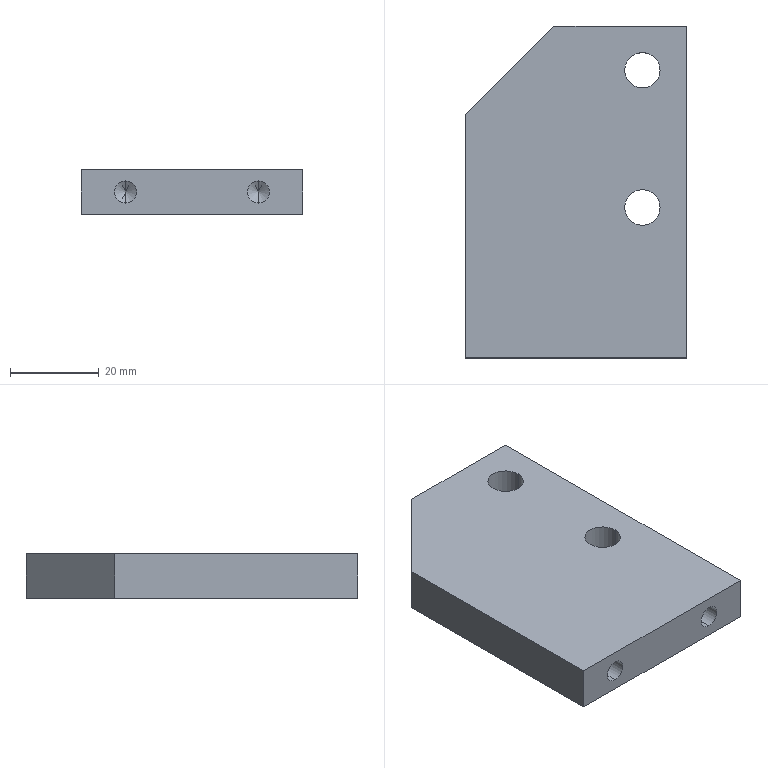Component | SolidWorks | JL001-05-05-002-1 | 1 solid | 19 faces | box 50 x 75 x 10 mm | volume 33886 mm3 | cylinder 8 | plane 7 | cone 4 | commonest cylinder face diameters 5 x4 8 x4
build123d program:
from build123d import *

# Parameters (mm, degrees)
SKETCH1_W             = 50
SKETCH1_H             = 75
BOSS_EXTRUDE1_DEPTH   = 5
M8X1_0_TAPPED_HOLE1_D = 8
M6_TAPPED_HOLE1_D     = 5
M6_TAPPED_HOLE1_DEPTH = 15
M6_TAPPED_HOLE1_TIP   = 1.502
CHAMFER1_SIZE         = 20


with BuildPart() as part:
    # Sketch1 → Boss-Extrude1 (new, symmetric)
    with BuildSketch(Plane.XY):
        Rectangle(SKETCH1_W, SKETCH1_H)
    extrude(amount=BOSS_EXTRUDE1_DEPTH, both=True)

    # M8x1.0 Tapped Hole1 (through all)
    with Locations(Plane.XY.offset(5)):
        with Locations((15, 27.5), (15, -3.5)):
            Hole(M8X1_0_TAPPED_HOLE1_D / 2)

    # M6 Tapped Hole1
    with Locations(Plane(origin=(0, -37.5, 0), x_dir=(-1, 0, 0), z_dir=(0, -1, 0))):
        with Locations((15, 0), (-15, 0)):
            Hole(M6_TAPPED_HOLE1_D / 2, depth=M6_TAPPED_HOLE1_DEPTH)
            with Locations((0, 0, -(M6_TAPPED_HOLE1_DEPTH + M6_TAPPED_HOLE1_TIP / 2))):  # 118° drill point
                Cone(0, M6_TAPPED_HOLE1_D / 2, M6_TAPPED_HOLE1_TIP, mode=Mode.SUBTRACT)

    # Chamfer1
    chamfer1_edges = [part.edges().sort_by_distance(p)[0] for p in [
        (-25, 37.5, 0),
    ]]
    chamfer(chamfer1_edges, length=CHAMFER1_SIZE)


solid = part.part

# Placed as in the assembly
solid = solid.moved(Location((0, 0, 137.5), (0, 0, 0)))
STEP:
#1=CARTESIAN_POINT('',(-0.5906,-0.8858,5.512));
#2=VERTEX_POINT('',#1);
#3=CARTESIAN_POINT('',(-0.5906,-0.8858,5.315));
#4=VERTEX_POINT('',#3);
#5=CARTESIAN_POINT('',(-0.5906,-0.8858,5.413));
#6=DIRECTION('',(0.,-1.,0.));
#7=DIRECTION('',(0.,0.,-1.));
#8=AXIS2_PLACEMENT_3D('',#5,#6,#7);
#9=CIRCLE('',#8,0.09843);
#10=EDGE_CURVE('',#2,#4,#9,.T.);
#11=ORIENTED_EDGE('',*,*,#10,.F.);
#12=CARTESIAN_POINT('',(-0.5906,-1.476,5.512));
#13=VERTEX_POINT('',#12);
#14=CARTESIAN_POINT('',(-0.5906,-1.476,5.512));
#15=DIRECTION('',(0.,-1.,0.));
#16=VECTOR('',#15,39.37);
#17=LINE('',#14,#16);
#18=EDGE_CURVE('',#2,#13,#17,.T.);
#19=ORIENTED_EDGE('',*,*,#18,.T.);
#20=CARTESIAN_POINT('',(-0.5906,-1.476,5.315));
#21=VERTEX_POINT('',#20);
#22=CARTESIAN_POINT('',(-0.5906,-1.476,5.413));
#23=DIRECTION('',(0.,-1.,0.));
#24=DIRECTION('',(0.,0.,-1.));
#25=AXIS2_PLACEMENT_3D('',#22,#23,#24);
#26=CIRCLE('',#25,0.09843);
#27=EDGE_CURVE('',#13,#21,#26,.T.);
#28=ORIENTED_EDGE('',*,*,#27,.T.);
#29=CARTESIAN_POINT('',(-0.5906,-1.476,5.315));
#30=DIRECTION('',(0.,-1.,0.));
#31=VECTOR('',#30,39.37);
#32=LINE('',#29,#31);
#33=EDGE_CURVE('',#4,#21,#32,.T.);
#34=ORIENTED_EDGE('',*,*,#33,.F.);
#35=EDGE_LOOP('',(#11,#19,#28,#34));
#36=FACE_OUTER_BOUND('',#35,.T.);
#37=CARTESIAN_POINT('',(-0.5906,-1.476,5.413));
#38=DIRECTION('',(0.,-1.,0.));
#39=DIRECTION('',(0.,0.,-1.));
#40=AXIS2_PLACEMENT_3D('',#37,#38,#39);
#41=CYLINDRICAL_SURFACE('',#40,0.09843);
#42=ADVANCED_FACE('',(#36),#41,.F.);
#43=CARTESIAN_POINT('',(-0.5906,-0.8267,5.413));
#44=VERTEX_POINT('',#43);
#45=CARTESIAN_POINT('',(-0.5906,-0.8858,5.315));
#46=DIRECTION('',(0.,-0.515,-0.8572));
#47=VECTOR('',#46,39.37);
#48=LINE('',#45,#47);
#49=EDGE_CURVE('',#44,#4,#48,.T.);
#50=ORIENTED_EDGE('',*,*,#49,.F.);
#51=CARTESIAN_POINT('',(-0.5906,-0.8858,5.512));
#52=DIRECTION('',(0.,-0.515,0.8572));
#53=VECTOR('',#52,39.37);
#54=LINE('',#51,#53);
#55=EDGE_CURVE('',#44,#2,#54,.T.);
#56=ORIENTED_EDGE('',*,*,#55,.T.);
#57=ORIENTED_EDGE('',*,*,#10,.T.);
#58=EDGE_LOOP('',(#50,#56,#57));
#59=FACE_OUTER_BOUND('',#58,.T.);
#60=CARTESIAN_POINT('',(-0.5906,-0.8858,5.413));
#61=DIRECTION('',(0.,-1.,0.));
#62=DIRECTION('',(0.,0.,-1.));
#63=AXIS2_PLACEMENT_3D('',#60,#61,#62);
#64=CONICAL_SURFACE('',#63,0.09843,1.03);
#65=ADVANCED_FACE('',(#59),#64,.F.);
#66=CARTESIAN_POINT('',(0.5906,-0.8858,5.512));
#67=VERTEX_POINT('',#66);
#68=CARTESIAN_POINT('',(0.5906,-0.8858,5.315));
#69=VERTEX_POINT('',#68);
#70=CARTESIAN_POINT('',(0.5906,-0.8858,5.413));
#71=DIRECTION('',(0.,-1.,0.));
#72=DIRECTION('',(0.,0.,-1.));
#73=AXIS2_PLACEMENT_3D('',#70,#71,#72);
#74=CIRCLE('',#73,0.09843);
#75=EDGE_CURVE('',#67,#69,#74,.T.);
#76=ORIENTED_EDGE('',*,*,#75,.F.);
#77=CARTESIAN_POINT('',(0.5906,-1.476,5.512));
#78=VERTEX_POINT('',#77);
#79=CARTESIAN_POINT('',(0.5906,-1.476,5.512));
#80=DIRECTION('',(0.,-1.,0.));
#81=VECTOR('',#80,39.37);
#82=LINE('',#79,#81);
#83=EDGE_CURVE('',#67,#78,#82,.T.);
#84=ORIENTED_EDGE('',*,*,#83,.T.);
#85=CARTESIAN_POINT('',(0.5906,-1.476,5.315));
#86=VERTEX_POINT('',#85);
#87=CARTESIAN_POINT('',(0.5906,-1.476,5.413));
#88=DIRECTION('',(0.,-1.,0.));
#89=DIRECTION('',(0.,0.,-1.));
#90=AXIS2_PLACEMENT_3D('',#87,#88,#89);
#91=CIRCLE('',#90,0.09843);
#92=EDGE_CURVE('',#78,#86,#91,.T.);
#93=ORIENTED_EDGE('',*,*,#92,.T.);
#94=CARTESIAN_POINT('',(0.5906,-1.476,5.315));
#95=DIRECTION('',(0.,-1.,0.));
#96=VECTOR('',#95,39.37);
#97=LINE('',#94,#96);
#98=EDGE_CURVE('',#69,#86,#97,.T.);
#99=ORIENTED_EDGE('',*,*,#98,.F.);
#100=EDGE_LOOP('',(#76,#84,#93,#99));
#101=FACE_OUTER_BOUND('',#100,.T.);
#102=CARTESIAN_POINT('',(0.5906,-1.476,5.413));
#103=DIRECTION('',(0.,-1.,0.));
#104=DIRECTION('',(0.,0.,-1.));
#105=AXIS2_PLACEMENT_3D('',#102,#103,#104);
#106=CYLINDRICAL_SURFACE('',#105,0.09843);
#107=ADVANCED_FACE('',(#101),#106,.F.);
#108=CARTESIAN_POINT('',(0.5906,-0.8267,5.413));
#109=VERTEX_POINT('',#108);
#110=CARTESIAN_POINT('',(0.5906,-0.8858,5.315));
#111=DIRECTION('',(0.,-0.515,-0.8572));
#112=VECTOR('',#111,39.37);
#113=LINE('',#110,#112);
#114=EDGE_CURVE('',#109,#69,#113,.T.);
#115=ORIENTED_EDGE('',*,*,#114,.F.);
#116=CARTESIAN_POINT('',(0.5906,-0.8858,5.512));
#117=DIRECTION('',(0.,-0.515,0.8572));
#118=VECTOR('',#117,39.37);
#119=LINE('',#116,#118);
#120=EDGE_CURVE('',#109,#67,#119,.T.);
#121=ORIENTED_EDGE('',*,*,#120,.T.);
#122=ORIENTED_EDGE('',*,*,#75,.T.);
#123=EDGE_LOOP('',(#115,#121,#122));
#124=FACE_OUTER_BOUND('',#123,.T.);
#125=CARTESIAN_POINT('',(0.5906,-0.8858,5.413));
#126=DIRECTION('',(0.,-1.,0.));
#127=DIRECTION('',(0.,0.,-1.));
#128=AXIS2_PLACEMENT_3D('',#125,#126,#127);
#129=CONICAL_SURFACE('',#128,0.09843,1.03);
#130=ADVANCED_FACE('',(#124),#129,.F.);
#131=CARTESIAN_POINT('',(0.4331,1.083,5.217));
#132=VERTEX_POINT('',#131);
#133=CARTESIAN_POINT('',(0.748,1.083,5.217));
#134=VERTEX_POINT('',#133);
#135=CARTESIAN_POINT('',(0.5906,1.083,5.217));
#136=DIRECTION('',(0.,0.,1.));
#137=DIRECTION('',(1.,0.,0.));
#138=AXIS2_PLACEMENT_3D('',#135,#136,#137);
#139=CIRCLE('',#138,0.1575);
#140=EDGE_CURVE('',#132,#134,#139,.T.);
#141=ORIENTED_EDGE('',*,*,#140,.F.);
#142=CARTESIAN_POINT('',(0.4331,1.083,5.61));
#143=VERTEX_POINT('',#142);
#144=CARTESIAN_POINT('',(0.4331,1.083,5.61));
#145=DIRECTION('',(0.,0.,1.));
#146=VECTOR('',#145,39.37);
#147=LINE('',#144,#146);
#148=EDGE_CURVE('',#132,#143,#147,.T.);
#149=ORIENTED_EDGE('',*,*,#148,.T.);
#150=CARTESIAN_POINT('',(0.748,1.083,5.61));
#151=VERTEX_POINT('',#150);
#152=CARTESIAN_POINT('',(0.5906,1.083,5.61));
#153=DIRECTION('',(0.,0.,1.));
#154=DIRECTION('',(1.,0.,0.));
#155=AXIS2_PLACEMENT_3D('',#152,#153,#154);
#156=CIRCLE('',#155,0.1575);
#157=EDGE_CURVE('',#143,#151,#156,.T.);
#158=ORIENTED_EDGE('',*,*,#157,.T.);
#159=CARTESIAN_POINT('',(0.748,1.083,5.61));
#160=DIRECTION('',(0.,0.,1.));
#161=VECTOR('',#160,39.37);
#162=LINE('',#159,#161);
#163=EDGE_CURVE('',#134,#151,#162,.T.);
#164=ORIENTED_EDGE('',*,*,#163,.F.);
#165=EDGE_LOOP('',(#141,#149,#158,#164));
#166=FACE_OUTER_BOUND('',#165,.T.);
#167=CARTESIAN_POINT('',(0.5906,1.083,5.61));
#168=DIRECTION('',(0.,0.,1.));
#169=DIRECTION('',(1.,0.,0.));
#170=AXIS2_PLACEMENT_3D('',#167,#168,#169);
#171=CYLINDRICAL_SURFACE('',#170,0.1575);
#172=ADVANCED_FACE('',(#166),#171,.F.);
#173=CARTESIAN_POINT('',(0.4331,-0.1378,5.217));
#174=VERTEX_POINT('',#173);
#175=CARTESIAN_POINT('',(0.748,-0.1378,5.217));
#176=VERTEX_POINT('',#175);
#177=CARTESIAN_POINT('',(0.5906,-0.1378,5.217));
#178=DIRECTION('',(0.,0.,1.));
#179=DIRECTION('',(1.,0.,0.));
#180=AXIS2_PLACEMENT_3D('',#177,#178,#179);
#181=CIRCLE('',#180,0.1575);
#182=EDGE_CURVE('',#174,#176,#181,.T.);
#183=ORIENTED_EDGE('',*,*,#182,.F.);
#184=CARTESIAN_POINT('',(0.4331,-0.1378,5.61));
#185=VERTEX_POINT('',#184);
#186=CARTESIAN_POINT('',(0.4331,-0.1378,5.61));
#187=DIRECTION('',(0.,0.,1.));
#188=VECTOR('',#187,39.37);
#189=LINE('',#186,#188);
#190=EDGE_CURVE('',#174,#185,#189,.T.);
#191=ORIENTED_EDGE('',*,*,#190,.T.);
#192=CARTESIAN_POINT('',(0.748,-0.1378,5.61));
#193=VERTEX_POINT('',#192);
#194=CARTESIAN_POINT('',(0.5906,-0.1378,5.61));
#195=DIRECTION('',(0.,0.,1.));
#196=DIRECTION('',(1.,0.,0.));
#197=AXIS2_PLACEMENT_3D('',#194,#195,#196);
#198=CIRCLE('',#197,0.1575);
#199=EDGE_CURVE('',#185,#193,#198,.T.);
#200=ORIENTED_EDGE('',*,*,#199,.T.);
#201=CARTESIAN_POINT('',(0.748,-0.1378,5.61));
#202=DIRECTION('',(0.,0.,1.));
#203=VECTOR('',#202,39.37);
#204=LINE('',#201,#203);
#205=EDGE_CURVE('',#176,#193,#204,.T.);
#206=ORIENTED_EDGE('',*,*,#205,.F.);
#207=EDGE_LOOP('',(#183,#191,#200,#206));
#208=FACE_OUTER_BOUND('',#207,.T.);
#209=CARTESIAN_POINT('',(0.5906,-0.1378,5.61));
#210=DIRECTION('',(0.,0.,1.));
#211=DIRECTION('',(1.,0.,0.));
#212=AXIS2_PLACEMENT_3D('',#209,#210,#211);
#213=CYLINDRICAL_SURFACE('',#212,0.1575);
#214=ADVANCED_FACE('',(#208),#213,.F.);
#215=CARTESIAN_POINT('',(0.9843,-1.476,5.217));
#216=VERTEX_POINT('',#215);
#217=CARTESIAN_POINT('',(0.9843,1.476,5.217));
#218=VERTEX_POINT('',#217);
#219=CARTESIAN_POINT('',(0.9843,1.476,5.217));
#220=DIRECTION('',(-0.,1.,0.));
#221=VECTOR('',#220,39.37);
#222=LINE('',#219,#221);
#223=EDGE_CURVE('',#216,#218,#222,.T.);
#224=ORIENTED_EDGE('',*,*,#223,.T.);
#225=CARTESIAN_POINT('',(0.9843,1.476,5.61));
#226=VERTEX_POINT('',#225);
#227=CARTESIAN_POINT('',(0.9843,1.476,5.61));
#228=DIRECTION('',(0.,0.,-1.));
#229=VECTOR('',#228,39.37);
#230=LINE('',#227,#229);
#231=EDGE_CURVE('',#226,#218,#230,.T.);
#232=ORIENTED_EDGE('',*,*,#231,.F.);
#233=CARTESIAN_POINT('',(0.9843,-1.476,5.61));
#234=VERTEX_POINT('',#233);
#235=CARTESIAN_POINT('',(0.9843,1.476,5.61));
#236=DIRECTION('',(-0.,1.,0.));
#237=VECTOR('',#236,39.37);
#238=LINE('',#235,#237);
#239=EDGE_CURVE('',#234,#226,#238,.T.);
#240=ORIENTED_EDGE('',*,*,#239,.F.);
#241=CARTESIAN_POINT('',(0.9843,-1.476,5.61));
#242=DIRECTION('',(0.,0.,-1.));
#243=VECTOR('',#242,39.37);
#244=LINE('',#241,#243);
#245=EDGE_CURVE('',#234,#216,#244,.T.);
#246=ORIENTED_EDGE('',*,*,#245,.T.);
#247=EDGE_LOOP('',(#224,#232,#240,#246));
#248=FACE_OUTER_BOUND('',#247,.T.);
#249=CARTESIAN_POINT('',(0.9843,1.476,5.61));
#250=DIRECTION('',(-1.,-0.,0.));
#251=DIRECTION('',(0.,-1.,0.));
#252=AXIS2_PLACEMENT_3D('',#249,#250,#251);
#253=PLANE('',#252);
#254=ADVANCED_FACE('',(#248),#253,.F.);
#255=CARTESIAN_POINT('',(-0.1969,1.476,5.217));
#256=VERTEX_POINT('',#255);
#257=CARTESIAN_POINT('',(-0.9843,1.476,5.217));
#258=DIRECTION('',(-1.,0.,0.));
#259=VECTOR('',#258,39.37);
#260=LINE('',#257,#259);
#261=EDGE_CURVE('',#218,#256,#260,.T.);
#262=ORIENTED_EDGE('',*,*,#261,.T.);
#263=CARTESIAN_POINT('',(-0.1969,1.476,5.61));
#264=VERTEX_POINT('',#263);
#265=CARTESIAN_POINT('',(-0.1969,1.476,5.61));
#266=DIRECTION('',(0.,0.,1.));
#267=VECTOR('',#266,39.37);
#268=LINE('',#265,#267);
#269=EDGE_CURVE('',#256,#264,#268,.T.);
#270=ORIENTED_EDGE('',*,*,#269,.T.);
#271=CARTESIAN_POINT('',(-0.9843,1.476,5.61));
#272=DIRECTION('',(-1.,0.,0.));
#273=VECTOR('',#272,39.37);
#274=LINE('',#271,#273);
#275=EDGE_CURVE('',#226,#264,#274,.T.);
#276=ORIENTED_EDGE('',*,*,#275,.F.);
#277=ORIENTED_EDGE('',*,*,#231,.T.);
#278=EDGE_LOOP('',(#262,#270,#276,#277));
#279=FACE_OUTER_BOUND('',#278,.T.);
#280=CARTESIAN_POINT('',(-0.9843,1.476,5.61));
#281=DIRECTION('',(0.,-1.,0.));
#282=DIRECTION('',(0.,0.,-1.));
#283=AXIS2_PLACEMENT_3D('',#280,#281,#282);
#284=PLANE('',#283);
#285=ADVANCED_FACE('',(#279),#284,.F.);
#286=CARTESIAN_POINT('',(-0.9843,0.689,5.61));
#287=VERTEX_POINT('',#286);
#288=CARTESIAN_POINT('',(-0.9843,-1.476,5.61));
#289=VERTEX_POINT('',#288);
#290=CARTESIAN_POINT('',(-0.9843,1.476,5.61));
#291=DIRECTION('',(0.,-1.,0.));
#292=VECTOR('',#291,39.37);
#293=LINE('',#290,#292);
#294=EDGE_CURVE('',#287,#289,#293,.T.);
#295=ORIENTED_EDGE('',*,*,#294,.F.);
#296=CARTESIAN_POINT('',(-0.9843,0.689,5.217));
#297=VERTEX_POINT('',#296);
#298=CARTESIAN_POINT('',(-0.9843,0.689,5.61));
#299=DIRECTION('',(0.,0.,-1.));
#300=VECTOR('',#299,39.37);
#301=LINE('',#298,#300);
#302=EDGE_CURVE('',#287,#297,#301,.T.);
#303=ORIENTED_EDGE('',*,*,#302,.T.);
#304=CARTESIAN_POINT('',(-0.9843,-1.476,5.217));
#305=VERTEX_POINT('',#304);
#306=CARTESIAN_POINT('',(-0.9843,1.476,5.217));
#307=DIRECTION('',(0.,-1.,0.));
#308=VECTOR('',#307,39.37);
#309=LINE('',#306,#308);
#310=EDGE_CURVE('',#297,#305,#309,.T.);
#311=ORIENTED_EDGE('',*,*,#310,.T.);
#312=CARTESIAN_POINT('',(-0.9843,-1.476,5.61));
#313=DIRECTION('',(0.,0.,-1.));
#314=VECTOR('',#313,39.37);
#315=LINE('',#312,#314);
#316=EDGE_CURVE('',#289,#305,#315,.T.);
#317=ORIENTED_EDGE('',*,*,#316,.F.);
#318=EDGE_LOOP('',(#295,#303,#311,#317));
#319=FACE_OUTER_BOUND('',#318,.T.);
#320=CARTESIAN_POINT('',(-0.9843,1.476,5.61));
#321=DIRECTION('',(1.,0.,0.));
#322=DIRECTION('',(-0.,1.,0.));
#323=AXIS2_PLACEMENT_3D('',#320,#321,#322);
#324=PLANE('',#323);
#325=ADVANCED_FACE('',(#319),#324,.F.);
#326=CARTESIAN_POINT('',(-0.5906,-1.476,5.413));
#327=DIRECTION('',(0.,-1.,0.));
#328=DIRECTION('',(0.,0.,-1.));
#329=AXIS2_PLACEMENT_3D('',#326,#327,#328);
#330=CIRCLE('',#329,0.09843);
#331=EDGE_CURVE('',#21,#13,#330,.T.);
#332=ORIENTED_EDGE('',*,*,#331,.F.);
#333=ORIENTED_EDGE('',*,*,#27,.F.);
#334=EDGE_LOOP('',(#332,#333));
#335=FACE_BOUND('',#334,.T.);
#336=CARTESIAN_POINT('',(0.5906,-1.476,5.413));
#337=DIRECTION('',(0.,-1.,0.));
#338=DIRECTION('',(0.,0.,-1.));
#339=AXIS2_PLACEMENT_3D('',#336,#337,#338);
#340=CIRCLE('',#339,0.09843);
#341=EDGE_CURVE('',#86,#78,#340,.T.);
#342=ORIENTED_EDGE('',*,*,#341,.F.);
#343=ORIENTED_EDGE('',*,*,#92,.F.);
#344=EDGE_LOOP('',(#342,#343));
#345=FACE_BOUND('',#344,.T.);
#346=CARTESIAN_POINT('',(-0.9843,-1.476,5.217));
#347=DIRECTION('',(1.,0.,0.));
#348=VECTOR('',#347,39.37);
#349=LINE('',#346,#348);
#350=EDGE_CURVE('',#305,#216,#349,.T.);
#351=ORIENTED_EDGE('',*,*,#350,.T.);
#352=ORIENTED_EDGE('',*,*,#245,.F.);
#353=CARTESIAN_POINT('',(-0.9843,-1.476,5.61));
#354=DIRECTION('',(1.,0.,0.));
#355=VECTOR('',#354,39.37);
#356=LINE('',#353,#355);
#357=EDGE_CURVE('',#289,#234,#356,.T.);
#358=ORIENTED_EDGE('',*,*,#357,.F.);
#359=ORIENTED_EDGE('',*,*,#316,.T.);
#360=EDGE_LOOP('',(#351,#352,#358,#359));
#361=FACE_OUTER_BOUND('',#360,.T.);
#362=CARTESIAN_POINT('',(-0.9843,-1.476,5.61));
#363=DIRECTION('',(0.,1.,0.));
#364=DIRECTION('',(0.,0.,1.));
#365=AXIS2_PLACEMENT_3D('',#362,#363,#364);
#366=PLANE('',#365);
#367=ADVANCED_FACE('',(#335,#345,#361),#366,.F.);
#368=CARTESIAN_POINT('',(0.5906,1.083,5.61));
#369=DIRECTION('',(0.,0.,1.));
#370=DIRECTION('',(1.,0.,0.));
#371=AXIS2_PLACEMENT_3D('',#368,#369,#370);
#372=CIRCLE('',#371,0.1575);
#373=EDGE_CURVE('',#151,#143,#372,.T.);
#374=ORIENTED_EDGE('',*,*,#373,.F.);
#375=ORIENTED_EDGE('',*,*,#157,.F.);
#376=EDGE_LOOP('',(#374,#375));
#377=FACE_BOUND('',#376,.T.);
#378=CARTESIAN_POINT('',(0.5906,-0.1378,5.61));
#379=DIRECTION('',(0.,0.,1.));
#380=DIRECTION('',(1.,0.,0.));
#381=AXIS2_PLACEMENT_3D('',#378,#379,#380);
#382=CIRCLE('',#381,0.1575);
#383=EDGE_CURVE('',#193,#185,#382,.T.);
#384=ORIENTED_EDGE('',*,*,#383,.F.);
#385=ORIENTED_EDGE('',*,*,#199,.F.);
#386=EDGE_LOOP('',(#384,#385));
#387=FACE_BOUND('',#386,.T.);
#388=ORIENTED_EDGE('',*,*,#275,.T.);
#389=CARTESIAN_POINT('',(-0.8366,0.8366,5.61));
#390=DIRECTION('',(-0.7071,-0.7071,0.));
#391=VECTOR('',#390,39.37);
#392=LINE('',#389,#391);
#393=EDGE_CURVE('',#264,#287,#392,.T.);
#394=ORIENTED_EDGE('',*,*,#393,.T.);
#395=ORIENTED_EDGE('',*,*,#294,.T.);
#396=ORIENTED_EDGE('',*,*,#357,.T.);
#397=ORIENTED_EDGE('',*,*,#239,.T.);
#398=EDGE_LOOP('',(#388,#394,#395,#396,#397));
#399=FACE_OUTER_BOUND('',#398,.T.);
#400=CARTESIAN_POINT('',(0.,-0.,5.61));
#401=DIRECTION('',(0.,0.,1.));
#402=DIRECTION('',(1.,0.,0.));
#403=AXIS2_PLACEMENT_3D('',#400,#401,#402);
#404=PLANE('',#403);
#405=ADVANCED_FACE('',(#377,#387,#399),#404,.T.);
#406=CARTESIAN_POINT('',(0.5906,1.083,5.217));
#407=DIRECTION('',(0.,0.,1.));
#408=DIRECTION('',(1.,0.,0.));
#409=AXIS2_PLACEMENT_3D('',#406,#407,#408);
#410=CIRCLE('',#409,0.1575);
#411=EDGE_CURVE('',#134,#132,#410,.T.);
#412=ORIENTED_EDGE('',*,*,#411,.T.);
#413=ORIENTED_EDGE('',*,*,#140,.T.);
#414=EDGE_LOOP('',(#412,#413));
#415=FACE_BOUND('',#414,.T.);
#416=CARTESIAN_POINT('',(0.5906,-0.1378,5.217));
#417=DIRECTION('',(0.,0.,1.));
#418=DIRECTION('',(1.,0.,0.));
#419=AXIS2_PLACEMENT_3D('',#416,#417,#418);
#420=CIRCLE('',#419,0.1575);
#421=EDGE_CURVE('',#176,#174,#420,.T.);
#422=ORIENTED_EDGE('',*,*,#421,.T.);
#423=ORIENTED_EDGE('',*,*,#182,.T.);
#424=EDGE_LOOP('',(#422,#423));
#425=FACE_BOUND('',#424,.T.);
#426=ORIENTED_EDGE('',*,*,#310,.F.);
#427=CARTESIAN_POINT('',(-0.9843,0.689,5.217));
#428=DIRECTION('',(0.7071,0.7071,0.));
#429=VECTOR('',#428,39.37);
#430=LINE('',#427,#429);
#431=EDGE_CURVE('',#297,#256,#430,.T.);
#432=ORIENTED_EDGE('',*,*,#431,.T.);
#433=ORIENTED_EDGE('',*,*,#261,.F.);
#434=ORIENTED_EDGE('',*,*,#223,.F.);
#435=ORIENTED_EDGE('',*,*,#350,.F.);
#436=EDGE_LOOP('',(#426,#432,#433,#434,#435));
#437=FACE_OUTER_BOUND('',#436,.T.);
#438=CARTESIAN_POINT('',(0.,-0.,5.217));
#439=DIRECTION('',(0.,0.,1.));
#440=DIRECTION('',(1.,0.,0.));
#441=AXIS2_PLACEMENT_3D('',#438,#439,#440);
#442=PLANE('',#441);
#443=ADVANCED_FACE('',(#415,#425,#437),#442,.F.);
#444=ORIENTED_EDGE('',*,*,#190,.F.);
#445=ORIENTED_EDGE('',*,*,#421,.F.);
#446=ORIENTED_EDGE('',*,*,#205,.T.);
#447=ORIENTED_EDGE('',*,*,#383,.T.);
#448=EDGE_LOOP('',(#444,#445,#446,#447));
#449=FACE_OUTER_BOUND('',#448,.T.);
#450=CARTESIAN_POINT('',(0.5906,-0.1378,5.61));
#451=DIRECTION('',(0.,0.,1.));
#452=DIRECTION('',(1.,0.,0.));
#453=AXIS2_PLACEMENT_3D('',#450,#451,#452);
#454=CYLINDRICAL_SURFACE('',#453,0.1575);
#455=ADVANCED_FACE('',(#449),#454,.F.);
#456=ORIENTED_EDGE('',*,*,#148,.F.);
#457=ORIENTED_EDGE('',*,*,#411,.F.);
#458=ORIENTED_EDGE('',*,*,#163,.T.);
#459=ORIENTED_EDGE('',*,*,#373,.T.);
#460=EDGE_LOOP('',(#456,#457,#458,#459));
#461=FACE_OUTER_BOUND('',#460,.T.);
#462=CARTESIAN_POINT('',(0.5906,1.083,5.61));
#463=DIRECTION('',(0.,0.,1.));
#464=DIRECTION('',(1.,0.,0.));
#465=AXIS2_PLACEMENT_3D('',#462,#463,#464);
#466=CYLINDRICAL_SURFACE('',#465,0.1575);
#467=ADVANCED_FACE('',(#461),#466,.F.);
#468=ORIENTED_EDGE('',*,*,#120,.F.);
#469=ORIENTED_EDGE('',*,*,#114,.T.);
#470=CARTESIAN_POINT('',(0.5906,-0.8858,5.413));
#471=DIRECTION('',(0.,-1.,0.));
#472=DIRECTION('',(0.,0.,-1.));
#473=AXIS2_PLACEMENT_3D('',#470,#471,#472);
#474=CIRCLE('',#473,0.09843);
#475=EDGE_CURVE('',#69,#67,#474,.T.);
#476=ORIENTED_EDGE('',*,*,#475,.T.);
#477=EDGE_LOOP('',(#468,#469,#476));
#478=FACE_OUTER_BOUND('',#477,.T.);
#479=CARTESIAN_POINT('',(0.5906,-0.8858,5.413));
#480=DIRECTION('',(0.,-1.,0.));
#481=DIRECTION('',(0.,0.,-1.));
#482=AXIS2_PLACEMENT_3D('',#479,#480,#481);
#483=CONICAL_SURFACE('',#482,0.09843,1.03);
#484=ADVANCED_FACE('',(#478),#483,.F.);
#485=ORIENTED_EDGE('',*,*,#83,.F.);
#486=ORIENTED_EDGE('',*,*,#475,.F.);
#487=ORIENTED_EDGE('',*,*,#98,.T.);
#488=ORIENTED_EDGE('',*,*,#341,.T.);
#489=EDGE_LOOP('',(#485,#486,#487,#488));
#490=FACE_OUTER_BOUND('',#489,.T.);
#491=CARTESIAN_POINT('',(0.5906,-1.476,5.413));
#492=DIRECTION('',(0.,-1.,0.));
#493=DIRECTION('',(0.,0.,-1.));
#494=AXIS2_PLACEMENT_3D('',#491,#492,#493);
#495=CYLINDRICAL_SURFACE('',#494,0.09843);
#496=ADVANCED_FACE('',(#490),#495,.F.);
#497=ORIENTED_EDGE('',*,*,#55,.F.);
#498=ORIENTED_EDGE('',*,*,#49,.T.);
#499=CARTESIAN_POINT('',(-0.5906,-0.8858,5.413));
#500=DIRECTION('',(0.,-1.,0.));
#501=DIRECTION('',(0.,0.,-1.));
#502=AXIS2_PLACEMENT_3D('',#499,#500,#501);
#503=CIRCLE('',#502,0.09843);
#504=EDGE_CURVE('',#4,#2,#503,.T.);
#505=ORIENTED_EDGE('',*,*,#504,.T.);
#506=EDGE_LOOP('',(#497,#498,#505));
#507=FACE_OUTER_BOUND('',#506,.T.);
#508=CARTESIAN_POINT('',(-0.5906,-0.8858,5.413));
#509=DIRECTION('',(0.,-1.,0.));
#510=DIRECTION('',(0.,0.,-1.));
#511=AXIS2_PLACEMENT_3D('',#508,#509,#510);
#512=CONICAL_SURFACE('',#511,0.09843,1.03);
#513=ADVANCED_FACE('',(#507),#512,.F.);
#514=ORIENTED_EDGE('',*,*,#18,.F.);
#515=ORIENTED_EDGE('',*,*,#504,.F.);
#516=ORIENTED_EDGE('',*,*,#33,.T.);
#517=ORIENTED_EDGE('',*,*,#331,.T.);
#518=EDGE_LOOP('',(#514,#515,#516,#517));
#519=FACE_OUTER_BOUND('',#518,.T.);
#520=CARTESIAN_POINT('',(-0.5906,-1.476,5.413));
#521=DIRECTION('',(0.,-1.,0.));
#522=DIRECTION('',(0.,0.,-1.));
#523=AXIS2_PLACEMENT_3D('',#520,#521,#522);
#524=CYLINDRICAL_SURFACE('',#523,0.09843);
#525=ADVANCED_FACE('',(#519),#524,.F.);
#526=ORIENTED_EDGE('',*,*,#393,.F.);
#527=ORIENTED_EDGE('',*,*,#269,.F.);
#528=ORIENTED_EDGE('',*,*,#431,.F.);
#529=ORIENTED_EDGE('',*,*,#302,.F.);
#530=EDGE_LOOP('',(#526,#527,#528,#529));
#531=FACE_OUTER_BOUND('',#530,.T.);
#532=CARTESIAN_POINT('',(-0.9843,0.689,5.61));
#533=DIRECTION('',(0.7071,-0.7071,0.));
#534=DIRECTION('',(0.,0.,-1.));
#535=AXIS2_PLACEMENT_3D('',#532,#533,#534);
#536=PLANE('',#535);
#537=ADVANCED_FACE('',(#531),#536,.F.);
#538=CLOSED_SHELL('',(#42,#65,#107,#130,#172,#214,#254,#285,#325,#367,#405,#443,#455,#467,#484,#496,#513,#525,#537));
#539=MANIFOLD_SOLID_BREP('',#538);
#540=CARTESIAN_POINT('',(0.,0.,0.));
#541=DIRECTION('',(0.,0.,1.));
#542=DIRECTION('',(1.,0.,0.));
#543=AXIS2_PLACEMENT_3D('',#540,#541,#542);
#544=(LENGTH_UNIT()NAMED_UNIT(*)SI_UNIT($,.METRE.));
#545=LENGTH_MEASURE_WITH_UNIT(LENGTH_MEASURE(0.0254),#544);
#546=DIMENSIONAL_EXPONENTS(1.,0.,0.,0.,0.,0.,0.);
#547=(CONVERSION_BASED_UNIT('',#545)LENGTH_UNIT()NAMED_UNIT(#546));
#548=UNCERTAINTY_MEASURE_WITH_UNIT(LENGTH_MEASURE(0.00001),#547,'','');
#549=(NAMED_UNIT(*)PLANE_ANGLE_UNIT()SI_UNIT($,.RADIAN.));
#550=(NAMED_UNIT(*)SI_UNIT($,.STERADIAN.)SOLID_ANGLE_UNIT());
#551=(GEOMETRIC_REPRESENTATION_CONTEXT(3)GLOBAL_UNCERTAINTY_ASSIGNED_CONTEXT((#548))GLOBAL_UNIT_ASSIGNED_CONTEXT((#547,#549,#550))REPRESENTATION_CONTEXT('',''));
#552=ADVANCED_BREP_SHAPE_REPRESENTATION('',(#539,#543),#551);
#553=COLOUR_RGB('',0.7922,0.8196,0.9333);
#554=FILL_AREA_STYLE_COLOUR('',#553);
#555=FILL_AREA_STYLE('',(#554));
#556=SURFACE_STYLE_FILL_AREA(#555);
#557=SURFACE_SIDE_STYLE('',(#556));
#558=SURFACE_STYLE_USAGE(.BOTH.,#557);
#559=PRESENTATION_STYLE_ASSIGNMENT((#558));
#560=STYLED_ITEM('',(#559),#539);
#561=(LENGTH_UNIT()NAMED_UNIT(*)SI_UNIT($,.METRE.));
#562=LENGTH_MEASURE_WITH_UNIT(LENGTH_MEASURE(0.0254),#561);
#563=DIMENSIONAL_EXPONENTS(1.,0.,0.,0.,0.,0.,0.);
#564=(CONVERSION_BASED_UNIT('',#562)LENGTH_UNIT()NAMED_UNIT(#563));
#565=UNCERTAINTY_MEASURE_WITH_UNIT(LENGTH_MEASURE(0.00001),#564,'','');
#566=(NAMED_UNIT(*)PLANE_ANGLE_UNIT()SI_UNIT($,.RADIAN.));
#567=(NAMED_UNIT(*)SI_UNIT($,.STERADIAN.)SOLID_ANGLE_UNIT());
#568=(GEOMETRIC_REPRESENTATION_CONTEXT(3)GLOBAL_UNCERTAINTY_ASSIGNED_CONTEXT((#565))GLOBAL_UNIT_ASSIGNED_CONTEXT((#564,#566,#567))REPRESENTATION_CONTEXT('',''));
#569=MECHANICAL_DESIGN_GEOMETRIC_PRESENTATION_REPRESENTATION('',(#560),#568);
#570=PRESENTATION_LAYER_ASSIGNMENT('','',(#560));